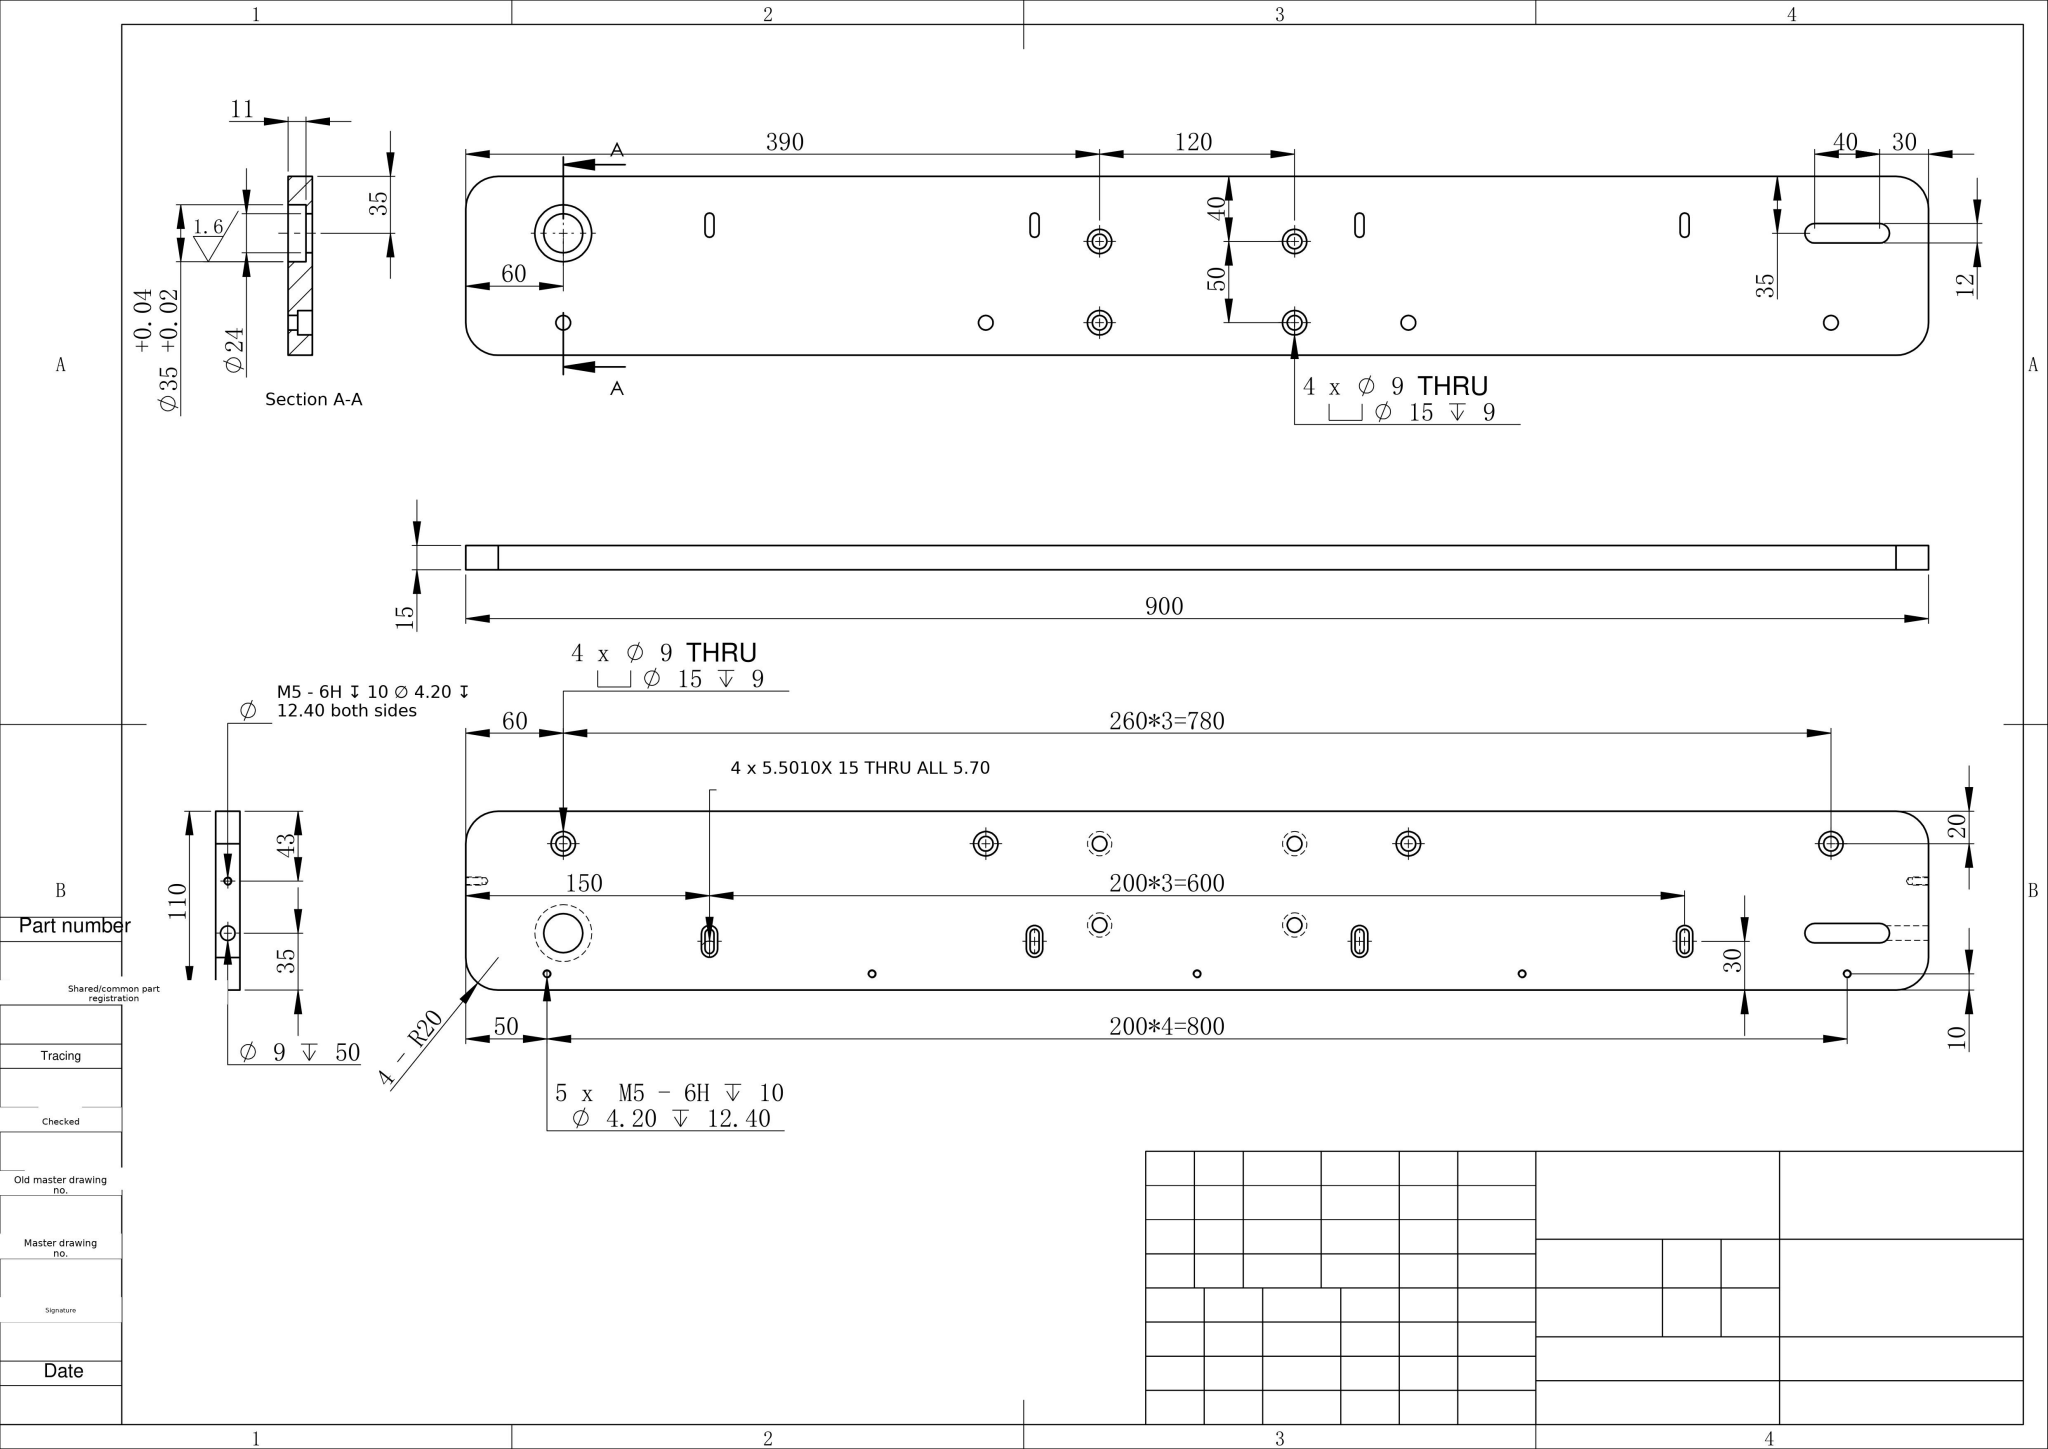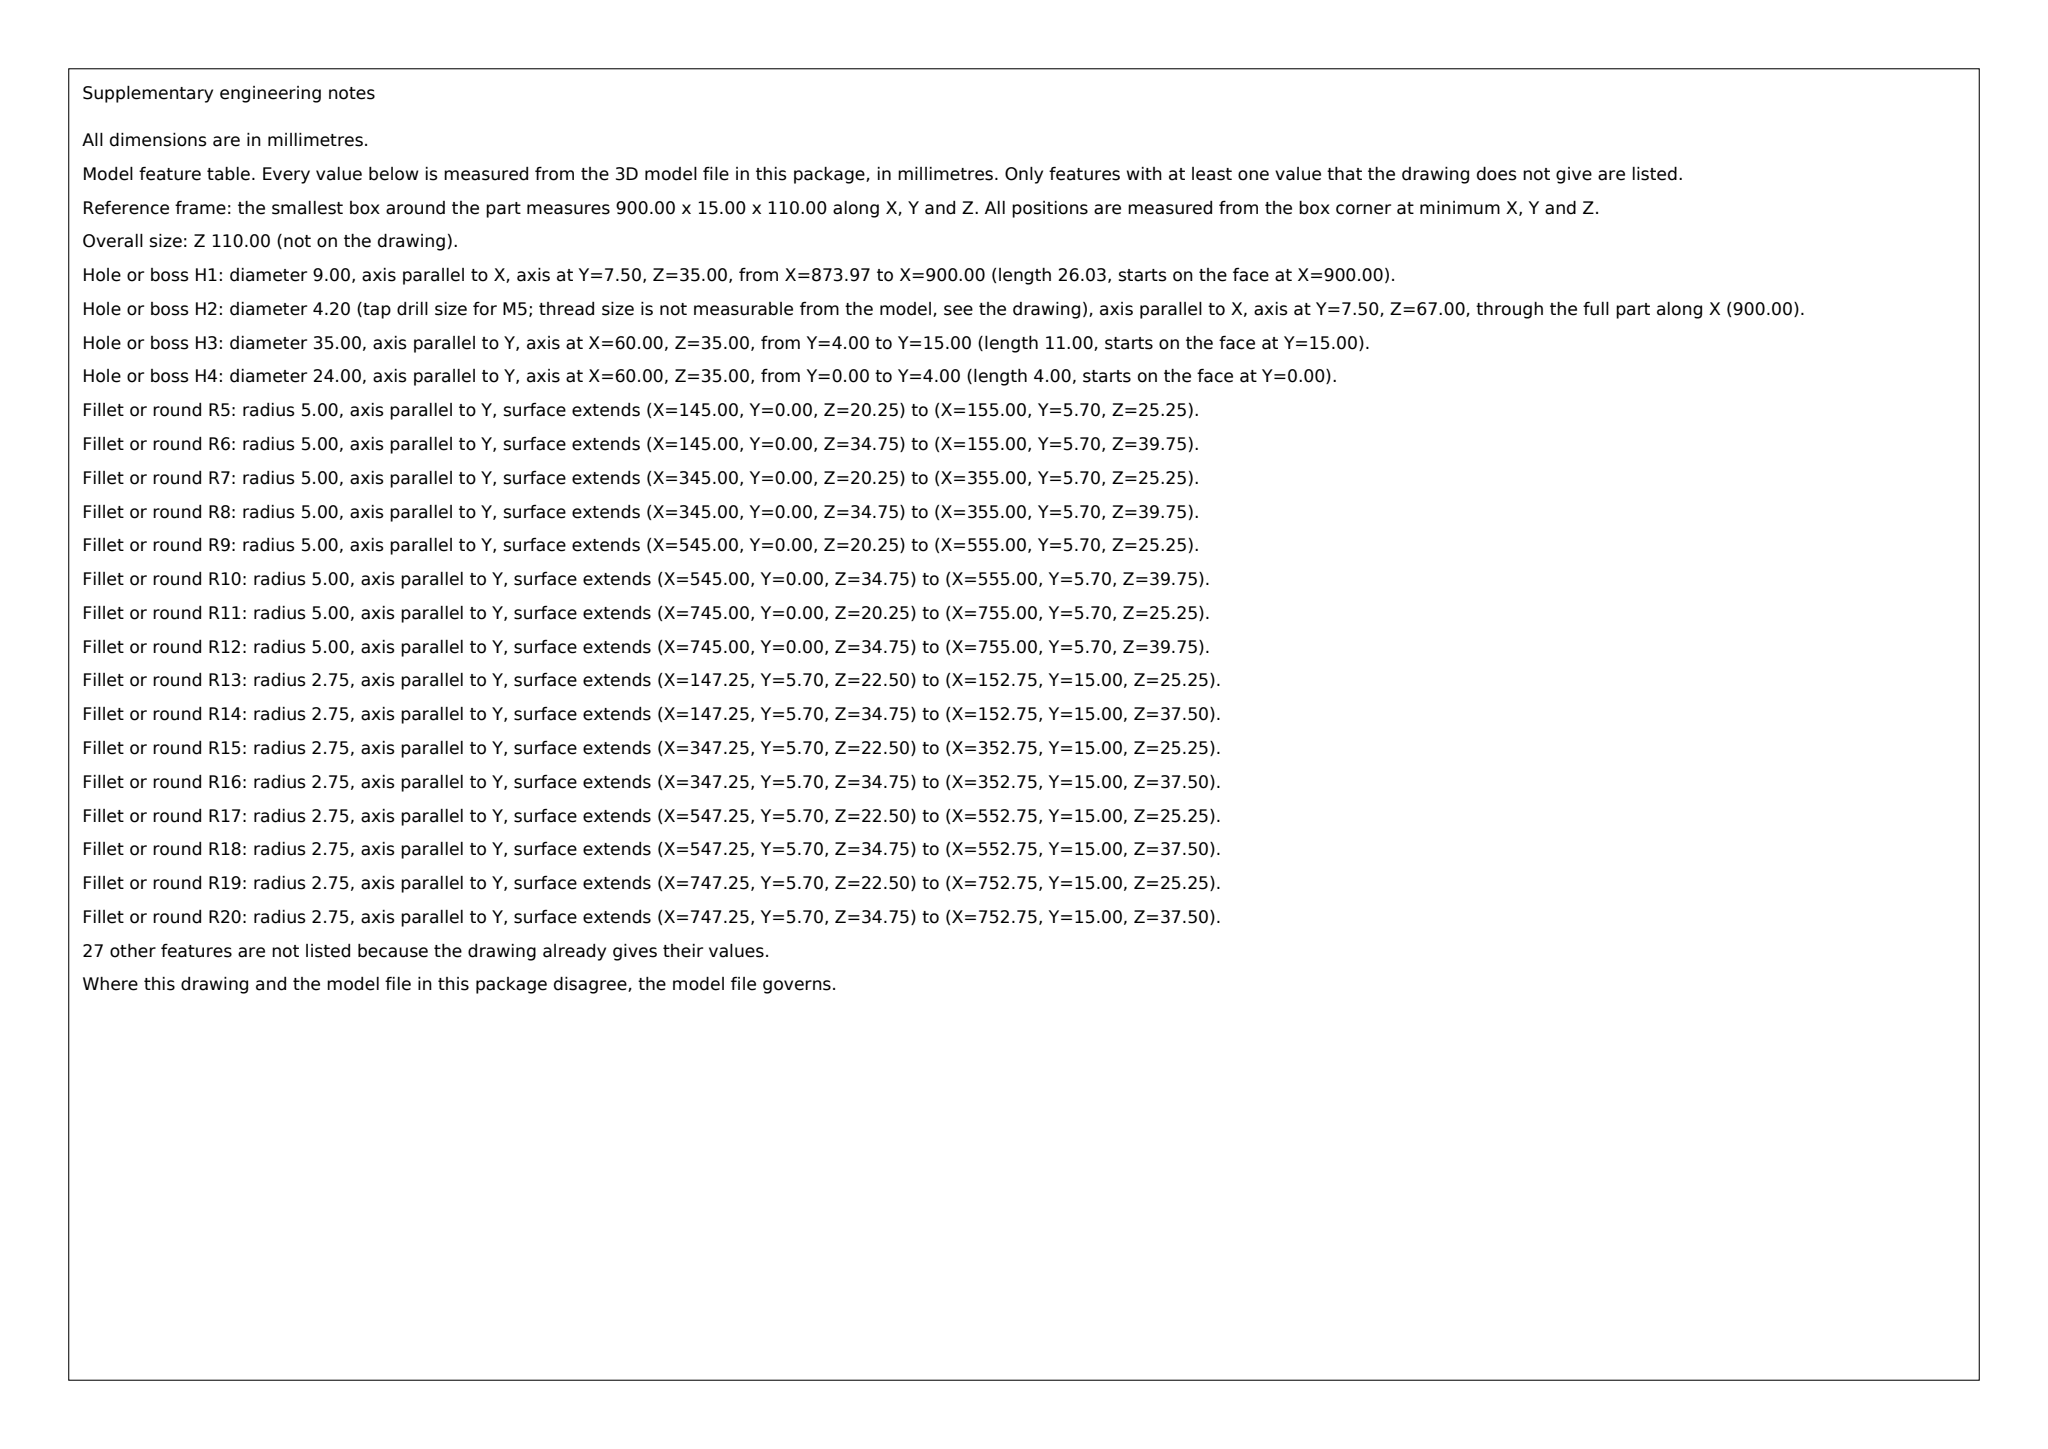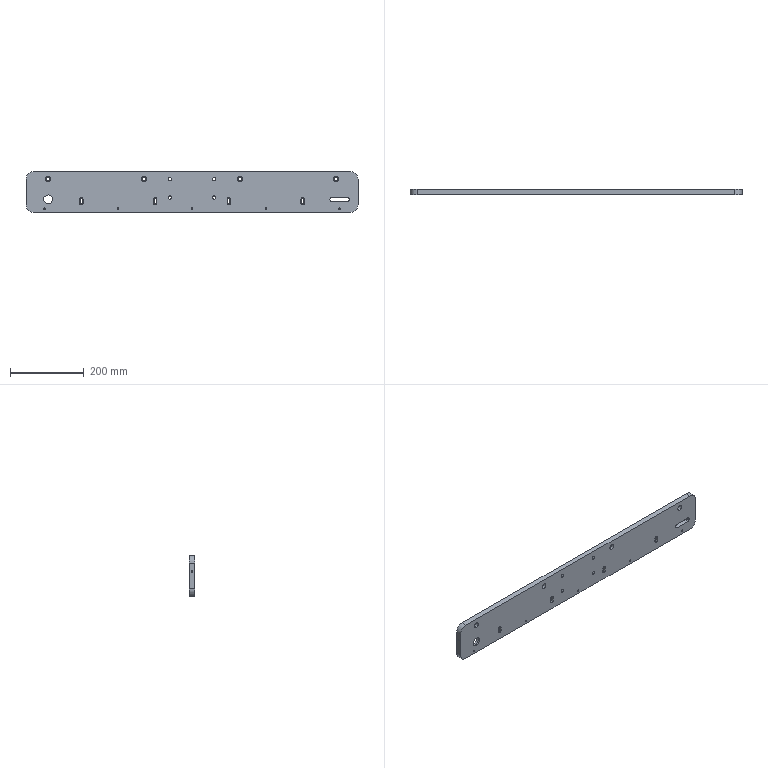Part | SolidWorks | mm | 1 solid | 133 faces | box 900 x 15 x 110 mm | volume 1433200 mm3 | cylinder 82 | plane 37 | cone 14 | commonest cylinder face diameters 9 x18 15 x16 4.2 x14 10 x12 5.5 x12 40 x4 24 x2 35 x2